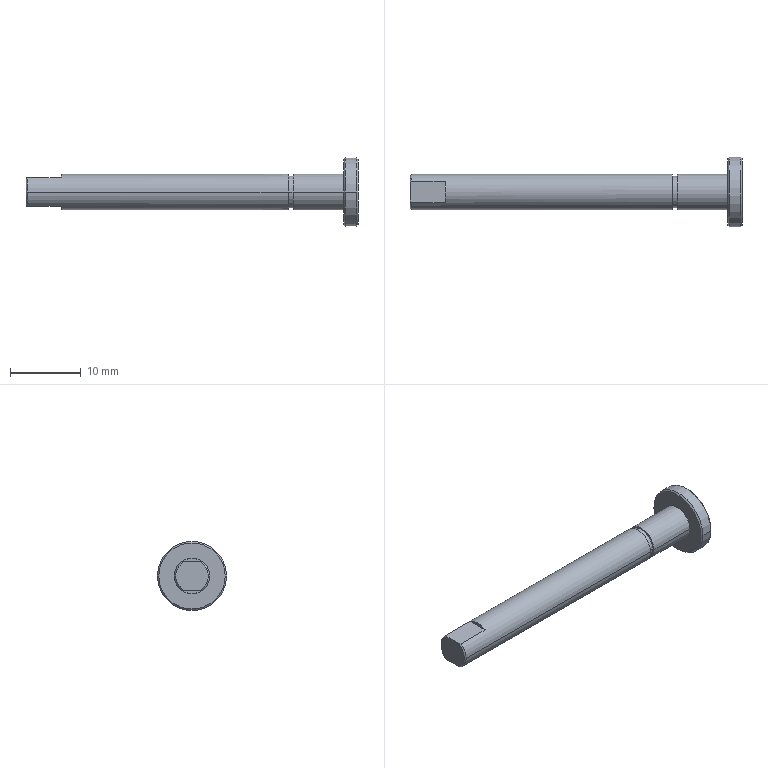Component | SolidWorks | 18MTOSC80BatteryCellCornerFoldingRollerAssembly-1_18ZTJ-NVT-01-002-1 | 1 solid | 24 faces | box 47 x 9.8 x 9.8 mm | volume 1020 mm3 | plane 9 | cylinder 8 | cone 7 | commonest cylinder face diameters 5 x4 4.5 x2 9.8 x2 | material Chrome Plated Rod
build123d program:
from build123d import *

# Parameters (mm, degrees)
SKETCH1_R           = 2.5
BOSS_EXTRUDE1_DEPTH = 45
SKETCH2_R           = 4.9
BOSS_EXTRUDE2_DEPTH = 2
CHAMFER1_SIZE       = 0.2
CUT_EXTRUDE2_START  = 0.7
SKETCH4_R           = 2.5
SKETCH4_R_2         = 2.25
CUT_EXTRUDE2_DEPTH  = 0.7
CUT_EXTRUDE3_DEPTH  = 5


with BuildPart() as part:
    # Sketch1 → Boss-Extrude1 (new body)
    with BuildSketch(Plane(origin=(0, 0, 0), x_dir=(1, 0, 0), z_dir=(0, 1, 0))):
        with Locations(Location((0, 0, 0), (0, 0, 90))):
            Circle(SKETCH1_R)
    extrude(amount=BOSS_EXTRUDE1_DEPTH)

    # Sketch2 → Boss-Extrude2 (add)
    with BuildSketch(Plane(origin=(0, 45, 0), x_dir=(1, 0, 0), z_dir=(0, 1, 0))):
        with Locations(Location((0, 0, 0), (0, 0, 270))):
            Circle(SKETCH2_R)
    extrude(amount=BOSS_EXTRUDE2_DEPTH)

    # Chamfer1
    chamfer1_edges = [part.edges().sort_by_distance(p)[0] for p in [
        (0, 0, 2.5),
        (0, 45, -4.9),
        (0, 47, -4.9),
    ]]
    chamfer(chamfer1_edges, length=CHAMFER1_SIZE)

    # Sketch4 → Cut-Extrude2 (cut)
    with BuildSketch(Plane(origin=(0, 37.8, 0), x_dir=(-1, 0, 0), z_dir=(0, -1, 0)).offset(CUT_EXTRUDE2_START)):
        with Locations(Location((0, 0, 0), (0, 0, 90))):
            Circle(SKETCH4_R)
        with Locations(Location((0, 0, 0), (0, 0, 90))):
            Circle(SKETCH4_R_2, mode=Mode.SUBTRACT)
    extrude(amount=-CUT_EXTRUDE2_DEPTH, mode=Mode.SUBTRACT)

    # Sketch5 → Cut-Extrude3 (cut)
    with BuildSketch(Plane.XZ):
        with BuildLine():
            Line((-2, 1.5), (-2, -1.5))
            ThreePointArc((-2, -1.5), (-2.5, 0), (-2, 1.5))
        make_face()
        with BuildLine():
            Line((2, 1.5), (2, -1.5))
            ThreePointArc((2, -1.5), (2.5, 0), (2, 1.5))
        make_face()
    extrude(amount=-CUT_EXTRUDE3_DEPTH, mode=Mode.SUBTRACT)


solid = part.part

# Placed as in the assembly
solid = solid.moved(Location((-30.1, -14.53, 131), (90, 0, -90)))
STEP:
#1=CARTESIAN_POINT('',(0.2756,-0.6705,5.157));
#2=VERTEX_POINT('',#1);
#3=CARTESIAN_POINT('',(0.2756,-0.4736,5.157));
#4=VERTEX_POINT('',#3);
#5=CARTESIAN_POINT('',(0.2756,-0.572,5.157));
#6=DIRECTION('',(-1.,-0.,-0.));
#7=DIRECTION('',(0.,-1.,0.));
#8=AXIS2_PLACEMENT_3D('',#5,#6,#7);
#9=CIRCLE('',#8,0.09843);
#10=EDGE_CURVE('',#2,#4,#9,.T.);
#11=ORIENTED_EDGE('',*,*,#10,.T.);
#12=CARTESIAN_POINT('',(-1.177,-0.4736,5.157));
#13=VERTEX_POINT('',#12);
#14=CARTESIAN_POINT('',(0.5866,-0.4736,5.157));
#15=DIRECTION('',(-1.,-0.,-0.));
#16=VECTOR('',#15,39.37);
#17=LINE('',#14,#16);
#18=EDGE_CURVE('',#4,#13,#17,.T.);
#19=ORIENTED_EDGE('',*,*,#18,.T.);
#20=CARTESIAN_POINT('',(-1.177,-0.513,5.236));
#21=VERTEX_POINT('',#20);
#22=CARTESIAN_POINT('',(-1.177,-0.572,5.157));
#23=DIRECTION('',(1.,0.,0.));
#24=DIRECTION('',(0.,1.,0.));
#25=AXIS2_PLACEMENT_3D('',#22,#23,#24);
#26=CIRCLE('',#25,0.09843);
#27=EDGE_CURVE('',#13,#21,#26,.T.);
#28=ORIENTED_EDGE('',*,*,#27,.T.);
#29=CARTESIAN_POINT('',(-0.9882,-0.513,5.236));
#30=VERTEX_POINT('',#29);
#31=CARTESIAN_POINT('',(-0.9882,-0.513,5.236));
#32=DIRECTION('',(-1.,-0.,-0.));
#33=VECTOR('',#32,39.37);
#34=LINE('',#31,#33);
#35=EDGE_CURVE('',#30,#21,#34,.T.);
#36=ORIENTED_EDGE('',*,*,#35,.F.);
#37=CARTESIAN_POINT('',(-0.9882,-0.6311,5.236));
#38=VERTEX_POINT('',#37);
#39=CARTESIAN_POINT('',(-0.9882,-0.572,5.157));
#40=DIRECTION('',(-1.,-0.,-0.));
#41=DIRECTION('',(0.,-1.,0.));
#42=AXIS2_PLACEMENT_3D('',#39,#40,#41);
#43=CIRCLE('',#42,0.09843);
#44=EDGE_CURVE('',#38,#30,#43,.T.);
#45=ORIENTED_EDGE('',*,*,#44,.F.);
#46=CARTESIAN_POINT('',(-1.177,-0.6311,5.236));
#47=VERTEX_POINT('',#46);
#48=CARTESIAN_POINT('',(-0.9882,-0.6311,5.236));
#49=DIRECTION('',(-1.,-0.,-0.));
#50=VECTOR('',#49,39.37);
#51=LINE('',#48,#50);
#52=EDGE_CURVE('',#38,#47,#51,.T.);
#53=ORIENTED_EDGE('',*,*,#52,.T.);
#54=CARTESIAN_POINT('',(-1.177,-0.6705,5.157));
#55=VERTEX_POINT('',#54);
#56=CARTESIAN_POINT('',(-1.177,-0.572,5.157));
#57=DIRECTION('',(1.,0.,0.));
#58=DIRECTION('',(0.,1.,0.));
#59=AXIS2_PLACEMENT_3D('',#56,#57,#58);
#60=CIRCLE('',#59,0.09843);
#61=EDGE_CURVE('',#47,#55,#60,.T.);
#62=ORIENTED_EDGE('',*,*,#61,.T.);
#63=CARTESIAN_POINT('',(0.5866,-0.6705,5.157));
#64=DIRECTION('',(-1.,-0.,-0.));
#65=VECTOR('',#64,39.37);
#66=LINE('',#63,#65);
#67=EDGE_CURVE('',#2,#55,#66,.T.);
#68=ORIENTED_EDGE('',*,*,#67,.F.);
#69=EDGE_LOOP('',(#11,#19,#28,#36,#45,#53,#62,#68));
#70=FACE_OUTER_BOUND('',#69,.T.);
#71=CARTESIAN_POINT('',(0.5866,-0.572,5.157));
#72=DIRECTION('',(-1.,-0.,-0.));
#73=DIRECTION('',(0.,-1.,0.));
#74=AXIS2_PLACEMENT_3D('',#71,#72,#73);
#75=CYLINDRICAL_SURFACE('',#74,0.09843);
#76=ADVANCED_FACE('',(#70),#75,.T.);
#77=CARTESIAN_POINT('',(-1.185,-0.4815,5.157));
#78=VERTEX_POINT('',#77);
#79=CARTESIAN_POINT('',(-1.185,-0.5273,5.079));
#80=VERTEX_POINT('',#79);
#81=CARTESIAN_POINT('',(-1.185,-0.572,5.157));
#82=DIRECTION('',(-1.,-0.,-0.));
#83=DIRECTION('',(0.,1.,0.));
#84=AXIS2_PLACEMENT_3D('',#81,#82,#83);
#85=CIRCLE('',#84,0.09055);
#86=EDGE_CURVE('',#78,#80,#85,.T.);
#87=ORIENTED_EDGE('',*,*,#86,.F.);
#88=CARTESIAN_POINT('',(-1.177,-0.4736,5.157));
#89=DIRECTION('',(0.7071,0.7071,0.));
#90=VECTOR('',#89,39.37);
#91=LINE('',#88,#90);
#92=EDGE_CURVE('',#78,#13,#91,.T.);
#93=ORIENTED_EDGE('',*,*,#92,.T.);
#94=CARTESIAN_POINT('',(-1.177,-0.513,5.079));
#95=VERTEX_POINT('',#94);
#96=CARTESIAN_POINT('',(-1.177,-0.572,5.157));
#97=DIRECTION('',(1.,0.,0.));
#98=DIRECTION('',(0.,1.,0.));
#99=AXIS2_PLACEMENT_3D('',#96,#97,#98);
#100=CIRCLE('',#99,0.09843);
#101=EDGE_CURVE('',#95,#13,#100,.T.);
#102=ORIENTED_EDGE('',*,*,#101,.F.);
#103=CARTESIAN_POINT('',(-1.185,-0.5273,5.079));
#104=CARTESIAN_POINT('',(-1.183,-0.5224,5.079));
#105=CARTESIAN_POINT('',(-1.18,-0.5176,5.079));
#106=CARTESIAN_POINT('',(-1.177,-0.513,5.079));
#107=B_SPLINE_CURVE_WITH_KNOTS('',3,(#103,#104,#105,#106),.UNSPECIFIED.,.F.,.F.,(4,4),(0.005045,0.005461),.UNSPECIFIED.);
#108=EDGE_CURVE('',#80,#95,#107,.T.);
#109=ORIENTED_EDGE('',*,*,#108,.F.);
#110=EDGE_LOOP('',(#87,#93,#102,#109));
#111=FACE_OUTER_BOUND('',#110,.T.);
#112=CARTESIAN_POINT('',(-1.177,-0.572,5.157));
#113=DIRECTION('',(1.,0.,0.));
#114=DIRECTION('',(0.,1.,0.));
#115=AXIS2_PLACEMENT_3D('',#112,#113,#114);
#116=CONICAL_SURFACE('',#115,0.09843,0.7854);
#117=ADVANCED_FACE('',(#111),#116,.T.);
#118=CARTESIAN_POINT('',(0.2756,-0.6606,5.157));
#119=VERTEX_POINT('',#118);
#120=CARTESIAN_POINT('',(0.2756,-0.4835,5.157));
#121=VERTEX_POINT('',#120);
#122=CARTESIAN_POINT('',(0.2756,-0.572,5.157));
#123=DIRECTION('',(-1.,-0.,-0.));
#124=DIRECTION('',(0.,-1.,0.));
#125=AXIS2_PLACEMENT_3D('',#122,#123,#124);
#126=CIRCLE('',#125,0.08858);
#127=EDGE_CURVE('',#119,#121,#126,.T.);
#128=ORIENTED_EDGE('',*,*,#127,.F.);
#129=CARTESIAN_POINT('',(0.3032,-0.6606,5.157));
#130=VERTEX_POINT('',#129);
#131=CARTESIAN_POINT('',(0.2756,-0.6606,5.157));
#132=DIRECTION('',(1.,0.,0.));
#133=VECTOR('',#132,39.37);
#134=LINE('',#131,#133);
#135=EDGE_CURVE('',#119,#130,#134,.T.);
#136=ORIENTED_EDGE('',*,*,#135,.T.);
#137=CARTESIAN_POINT('',(0.3032,-0.4835,5.157));
#138=VERTEX_POINT('',#137);
#139=CARTESIAN_POINT('',(0.3032,-0.572,5.157));
#140=DIRECTION('',(-1.,-0.,-0.));
#141=DIRECTION('',(0.,-1.,0.));
#142=AXIS2_PLACEMENT_3D('',#139,#140,#141);
#143=CIRCLE('',#142,0.08858);
#144=EDGE_CURVE('',#130,#138,#143,.T.);
#145=ORIENTED_EDGE('',*,*,#144,.T.);
#146=CARTESIAN_POINT('',(0.2756,-0.4835,5.157));
#147=DIRECTION('',(1.,0.,0.));
#148=VECTOR('',#147,39.37);
#149=LINE('',#146,#148);
#150=EDGE_CURVE('',#121,#138,#149,.T.);
#151=ORIENTED_EDGE('',*,*,#150,.F.);
#152=EDGE_LOOP('',(#128,#136,#145,#151));
#153=FACE_OUTER_BOUND('',#152,.T.);
#154=CARTESIAN_POINT('',(0.2756,-0.572,5.157));
#155=DIRECTION('',(1.,0.,0.));
#156=DIRECTION('',(0.,1.,0.));
#157=AXIS2_PLACEMENT_3D('',#154,#155,#156);
#158=CYLINDRICAL_SURFACE('',#157,0.08858);
#159=ADVANCED_FACE('',(#153),#158,.T.);
#160=CARTESIAN_POINT('',(0.6654,-0.387,5.157));
#161=VERTEX_POINT('',#160);
#162=CARTESIAN_POINT('',(0.6654,-0.7571,5.157));
#163=VERTEX_POINT('',#162);
#164=CARTESIAN_POINT('',(0.6654,-0.572,5.157));
#165=DIRECTION('',(1.,0.,0.));
#166=DIRECTION('',(0.,1.,0.));
#167=AXIS2_PLACEMENT_3D('',#164,#165,#166);
#168=CIRCLE('',#167,0.185);
#169=EDGE_CURVE('',#161,#163,#168,.T.);
#170=ORIENTED_EDGE('',*,*,#169,.F.);
#171=CARTESIAN_POINT('',(0.6575,-0.3791,5.157));
#172=VERTEX_POINT('',#171);
#173=CARTESIAN_POINT('',(0.6654,-0.387,5.157));
#174=DIRECTION('',(-0.7071,0.7071,0.));
#175=VECTOR('',#174,39.37);
#176=LINE('',#173,#175);
#177=EDGE_CURVE('',#161,#172,#176,.T.);
#178=ORIENTED_EDGE('',*,*,#177,.T.);
#179=CARTESIAN_POINT('',(0.6575,-0.765,5.157));
#180=VERTEX_POINT('',#179);
#181=CARTESIAN_POINT('',(0.6575,-0.572,5.157));
#182=DIRECTION('',(-1.,-0.,-0.));
#183=DIRECTION('',(0.,1.,0.));
#184=AXIS2_PLACEMENT_3D('',#181,#182,#183);
#185=CIRCLE('',#184,0.1929);
#186=EDGE_CURVE('',#180,#172,#185,.T.);
#187=ORIENTED_EDGE('',*,*,#186,.F.);
#188=CARTESIAN_POINT('',(0.6654,-0.7571,5.157));
#189=DIRECTION('',(-0.7071,-0.7071,-0.));
#190=VECTOR('',#189,39.37);
#191=LINE('',#188,#190);
#192=EDGE_CURVE('',#163,#180,#191,.T.);
#193=ORIENTED_EDGE('',*,*,#192,.F.);
#194=EDGE_LOOP('',(#170,#178,#187,#193));
#195=FACE_OUTER_BOUND('',#194,.T.);
#196=CARTESIAN_POINT('',(0.6654,-0.572,5.157));
#197=DIRECTION('',(-1.,-0.,-0.));
#198=DIRECTION('',(0.,-1.,0.));
#199=AXIS2_PLACEMENT_3D('',#196,#197,#198);
#200=CONICAL_SURFACE('',#199,0.185,0.7854);
#201=ADVANCED_FACE('',(#195),#200,.T.);
#202=CARTESIAN_POINT('',(0.5866,-0.7571,5.157));
#203=VERTEX_POINT('',#202);
#204=CARTESIAN_POINT('',(0.5866,-0.387,5.157));
#205=VERTEX_POINT('',#204);
#206=CARTESIAN_POINT('',(0.5866,-0.572,5.157));
#207=DIRECTION('',(-1.,-0.,-0.));
#208=DIRECTION('',(0.,1.,0.));
#209=AXIS2_PLACEMENT_3D('',#206,#207,#208);
#210=CIRCLE('',#209,0.185);
#211=EDGE_CURVE('',#203,#205,#210,.T.);
#212=ORIENTED_EDGE('',*,*,#211,.F.);
#213=CARTESIAN_POINT('',(0.5945,-0.765,5.157));
#214=VERTEX_POINT('',#213);
#215=CARTESIAN_POINT('',(0.5945,-0.765,5.157));
#216=DIRECTION('',(0.7071,-0.7071,0.));
#217=VECTOR('',#216,39.37);
#218=LINE('',#215,#217);
#219=EDGE_CURVE('',#203,#214,#218,.T.);
#220=ORIENTED_EDGE('',*,*,#219,.T.);
#221=CARTESIAN_POINT('',(0.5945,-0.3791,5.157));
#222=VERTEX_POINT('',#221);
#223=CARTESIAN_POINT('',(0.5945,-0.572,5.157));
#224=DIRECTION('',(1.,0.,0.));
#225=DIRECTION('',(-0.,1.,0.));
#226=AXIS2_PLACEMENT_3D('',#223,#224,#225);
#227=CIRCLE('',#226,0.1929);
#228=EDGE_CURVE('',#222,#214,#227,.T.);
#229=ORIENTED_EDGE('',*,*,#228,.F.);
#230=CARTESIAN_POINT('',(0.5945,-0.3791,5.157));
#231=DIRECTION('',(0.7071,0.7071,0.));
#232=VECTOR('',#231,39.37);
#233=LINE('',#230,#232);
#234=EDGE_CURVE('',#205,#222,#233,.T.);
#235=ORIENTED_EDGE('',*,*,#234,.F.);
#236=EDGE_LOOP('',(#212,#220,#229,#235));
#237=FACE_OUTER_BOUND('',#236,.T.);
#238=CARTESIAN_POINT('',(0.5945,-0.572,5.157));
#239=DIRECTION('',(1.,0.,0.));
#240=DIRECTION('',(-0.,1.,0.));
#241=AXIS2_PLACEMENT_3D('',#238,#239,#240);
#242=CONICAL_SURFACE('',#241,0.1929,0.7854);
#243=ADVANCED_FACE('',(#237),#242,.T.);
#244=ORIENTED_EDGE('',*,*,#186,.T.);
#245=CARTESIAN_POINT('',(0.6654,-0.3791,5.157));
#246=DIRECTION('',(-1.,-0.,-0.));
#247=VECTOR('',#246,39.37);
#248=LINE('',#245,#247);
#249=EDGE_CURVE('',#172,#222,#248,.T.);
#250=ORIENTED_EDGE('',*,*,#249,.T.);
#251=ORIENTED_EDGE('',*,*,#228,.T.);
#252=CARTESIAN_POINT('',(0.6654,-0.765,5.157));
#253=DIRECTION('',(-1.,-0.,-0.));
#254=VECTOR('',#253,39.37);
#255=LINE('',#252,#254);
#256=EDGE_CURVE('',#180,#214,#255,.T.);
#257=ORIENTED_EDGE('',*,*,#256,.F.);
#258=EDGE_LOOP('',(#244,#250,#251,#257));
#259=FACE_OUTER_BOUND('',#258,.T.);
#260=CARTESIAN_POINT('',(0.6654,-0.572,5.157));
#261=DIRECTION('',(-1.,-0.,-0.));
#262=DIRECTION('',(0.,-1.,0.));
#263=AXIS2_PLACEMENT_3D('',#260,#261,#262);
#264=CYLINDRICAL_SURFACE('',#263,0.1929);
#265=ADVANCED_FACE('',(#259),#264,.T.);
#266=CARTESIAN_POINT('',(0.5866,-0.4736,5.157));
#267=VERTEX_POINT('',#266);
#268=CARTESIAN_POINT('',(0.5866,-0.6705,5.157));
#269=VERTEX_POINT('',#268);
#270=CARTESIAN_POINT('',(0.5866,-0.572,5.157));
#271=DIRECTION('',(1.,0.,0.));
#272=DIRECTION('',(0.,1.,0.));
#273=AXIS2_PLACEMENT_3D('',#270,#271,#272);
#274=CIRCLE('',#273,0.09843);
#275=EDGE_CURVE('',#267,#269,#274,.T.);
#276=ORIENTED_EDGE('',*,*,#275,.F.);
#277=CARTESIAN_POINT('',(0.3032,-0.4736,5.157));
#278=VERTEX_POINT('',#277);
#279=CARTESIAN_POINT('',(0.5866,-0.4736,5.157));
#280=DIRECTION('',(-1.,-0.,-0.));
#281=VECTOR('',#280,39.37);
#282=LINE('',#279,#281);
#283=EDGE_CURVE('',#267,#278,#282,.T.);
#284=ORIENTED_EDGE('',*,*,#283,.T.);
#285=CARTESIAN_POINT('',(0.3032,-0.6705,5.157));
#286=VERTEX_POINT('',#285);
#287=CARTESIAN_POINT('',(0.3032,-0.572,5.157));
#288=DIRECTION('',(-1.,-0.,-0.));
#289=DIRECTION('',(0.,-1.,0.));
#290=AXIS2_PLACEMENT_3D('',#287,#288,#289);
#291=CIRCLE('',#290,0.09843);
#292=EDGE_CURVE('',#286,#278,#291,.T.);
#293=ORIENTED_EDGE('',*,*,#292,.F.);
#294=CARTESIAN_POINT('',(0.5866,-0.6705,5.157));
#295=DIRECTION('',(-1.,-0.,-0.));
#296=VECTOR('',#295,39.37);
#297=LINE('',#294,#296);
#298=EDGE_CURVE('',#269,#286,#297,.T.);
#299=ORIENTED_EDGE('',*,*,#298,.F.);
#300=EDGE_LOOP('',(#276,#284,#293,#299));
#301=FACE_OUTER_BOUND('',#300,.T.);
#302=CARTESIAN_POINT('',(0.5866,-0.572,5.157));
#303=DIRECTION('',(-1.,-0.,-0.));
#304=DIRECTION('',(0.,-1.,0.));
#305=AXIS2_PLACEMENT_3D('',#302,#303,#304);
#306=CYLINDRICAL_SURFACE('',#305,0.09843);
#307=ADVANCED_FACE('',(#301),#306,.T.);
#308=CARTESIAN_POINT('',(-1.177,-0.6311,5.079));
#309=VERTEX_POINT('',#308);
#310=CARTESIAN_POINT('',(-1.185,-0.6168,5.079));
#311=VERTEX_POINT('',#310);
#312=CARTESIAN_POINT('',(-1.177,-0.6311,5.079));
#313=CARTESIAN_POINT('',(-1.18,-0.6264,5.079));
#314=CARTESIAN_POINT('',(-1.183,-0.6216,5.079));
#315=CARTESIAN_POINT('',(-1.185,-0.6168,5.079));
#316=B_SPLINE_CURVE_WITH_KNOTS('',3,(#312,#313,#314,#315),.UNSPECIFIED.,.F.,.F.,(4,4),(0.002264,0.002682),.UNSPECIFIED.);
#317=EDGE_CURVE('',#309,#311,#316,.T.);
#318=ORIENTED_EDGE('',*,*,#317,.F.);
#319=CARTESIAN_POINT('',(-1.177,-0.572,5.157));
#320=DIRECTION('',(1.,0.,0.));
#321=DIRECTION('',(0.,1.,0.));
#322=AXIS2_PLACEMENT_3D('',#319,#320,#321);
#323=CIRCLE('',#322,0.09843);
#324=EDGE_CURVE('',#55,#309,#323,.T.);
#325=ORIENTED_EDGE('',*,*,#324,.F.);
#326=ORIENTED_EDGE('',*,*,#61,.F.);
#327=CARTESIAN_POINT('',(-1.185,-0.6168,5.236));
#328=VERTEX_POINT('',#327);
#329=CARTESIAN_POINT('',(-1.185,-0.6168,5.236));
#330=CARTESIAN_POINT('',(-1.183,-0.6217,5.236));
#331=CARTESIAN_POINT('',(-1.18,-0.6264,5.236));
#332=CARTESIAN_POINT('',(-1.177,-0.6311,5.236));
#333=B_SPLINE_CURVE_WITH_KNOTS('',3,(#329,#330,#331,#332),.UNSPECIFIED.,.F.,.F.,(4,4),(0.005045,0.005461),.UNSPECIFIED.);
#334=EDGE_CURVE('',#328,#47,#333,.T.);
#335=ORIENTED_EDGE('',*,*,#334,.F.);
#336=CARTESIAN_POINT('',(-1.185,-0.572,5.157));
#337=DIRECTION('',(-1.,-0.,-0.));
#338=DIRECTION('',(0.,1.,0.));
#339=AXIS2_PLACEMENT_3D('',#336,#337,#338);
#340=CIRCLE('',#339,0.09055);
#341=EDGE_CURVE('',#311,#328,#340,.T.);
#342=ORIENTED_EDGE('',*,*,#341,.F.);
#343=EDGE_LOOP('',(#318,#325,#326,#335,#342));
#344=FACE_OUTER_BOUND('',#343,.T.);
#345=CARTESIAN_POINT('',(-1.177,-0.572,5.157));
#346=DIRECTION('',(1.,0.,0.));
#347=DIRECTION('',(0.,1.,0.));
#348=AXIS2_PLACEMENT_3D('',#345,#346,#347);
#349=CONICAL_SURFACE('',#348,0.09843,0.7854);
#350=ADVANCED_FACE('',(#344),#349,.T.);
#351=ORIENTED_EDGE('',*,*,#283,.F.);
#352=CARTESIAN_POINT('',(0.5866,-0.572,5.157));
#353=DIRECTION('',(1.,0.,0.));
#354=DIRECTION('',(0.,1.,0.));
#355=AXIS2_PLACEMENT_3D('',#352,#353,#354);
#356=CIRCLE('',#355,0.09843);
#357=EDGE_CURVE('',#269,#267,#356,.T.);
#358=ORIENTED_EDGE('',*,*,#357,.F.);
#359=ORIENTED_EDGE('',*,*,#298,.T.);
#360=CARTESIAN_POINT('',(0.3032,-0.572,5.157));
#361=DIRECTION('',(-1.,-0.,-0.));
#362=DIRECTION('',(0.,-1.,0.));
#363=AXIS2_PLACEMENT_3D('',#360,#361,#362);
#364=CIRCLE('',#363,0.09843);
#365=EDGE_CURVE('',#278,#286,#364,.T.);
#366=ORIENTED_EDGE('',*,*,#365,.F.);
#367=EDGE_LOOP('',(#351,#358,#359,#366));
#368=FACE_OUTER_BOUND('',#367,.T.);
#369=CARTESIAN_POINT('',(0.5866,-0.572,5.157));
#370=DIRECTION('',(-1.,-0.,-0.));
#371=DIRECTION('',(0.,-1.,0.));
#372=AXIS2_PLACEMENT_3D('',#369,#370,#371);
#373=CYLINDRICAL_SURFACE('',#372,0.09843);
#374=ADVANCED_FACE('',(#368),#373,.T.);
#375=ORIENTED_EDGE('',*,*,#249,.F.);
#376=CARTESIAN_POINT('',(0.6575,-0.572,5.157));
#377=DIRECTION('',(-1.,-0.,-0.));
#378=DIRECTION('',(0.,1.,0.));
#379=AXIS2_PLACEMENT_3D('',#376,#377,#378);
#380=CIRCLE('',#379,0.1929);
#381=EDGE_CURVE('',#172,#180,#380,.T.);
#382=ORIENTED_EDGE('',*,*,#381,.T.);
#383=ORIENTED_EDGE('',*,*,#256,.T.);
#384=CARTESIAN_POINT('',(0.5945,-0.572,5.157));
#385=DIRECTION('',(1.,0.,0.));
#386=DIRECTION('',(-0.,1.,0.));
#387=AXIS2_PLACEMENT_3D('',#384,#385,#386);
#388=CIRCLE('',#387,0.1929);
#389=EDGE_CURVE('',#214,#222,#388,.T.);
#390=ORIENTED_EDGE('',*,*,#389,.T.);
#391=EDGE_LOOP('',(#375,#382,#383,#390));
#392=FACE_OUTER_BOUND('',#391,.T.);
#393=CARTESIAN_POINT('',(0.6654,-0.572,5.157));
#394=DIRECTION('',(-1.,-0.,-0.));
#395=DIRECTION('',(0.,-1.,0.));
#396=AXIS2_PLACEMENT_3D('',#393,#394,#395);
#397=CYLINDRICAL_SURFACE('',#396,0.1929);
#398=ADVANCED_FACE('',(#392),#397,.T.);
#399=CARTESIAN_POINT('',(0.6654,-0.572,5.157));
#400=DIRECTION('',(1.,0.,0.));
#401=DIRECTION('',(0.,1.,0.));
#402=AXIS2_PLACEMENT_3D('',#399,#400,#401);
#403=CIRCLE('',#402,0.185);
#404=EDGE_CURVE('',#163,#161,#403,.T.);
#405=ORIENTED_EDGE('',*,*,#404,.T.);
#406=ORIENTED_EDGE('',*,*,#169,.T.);
#407=EDGE_LOOP('',(#405,#406));
#408=FACE_OUTER_BOUND('',#407,.T.);
#409=CARTESIAN_POINT('',(0.6654,-0.572,5.157));
#410=DIRECTION('',(1.,0.,0.));
#411=DIRECTION('',(-0.,1.,-0.));
#412=AXIS2_PLACEMENT_3D('',#409,#410,#411);
#413=PLANE('',#412);
#414=ADVANCED_FACE('',(#408),#413,.T.);
#415=CARTESIAN_POINT('',(0.5866,-0.572,5.157));
#416=DIRECTION('',(-1.,-0.,-0.));
#417=DIRECTION('',(0.,1.,0.));
#418=AXIS2_PLACEMENT_3D('',#415,#416,#417);
#419=CIRCLE('',#418,0.185);
#420=EDGE_CURVE('',#205,#203,#419,.T.);
#421=ORIENTED_EDGE('',*,*,#420,.T.);
#422=ORIENTED_EDGE('',*,*,#211,.T.);
#423=EDGE_LOOP('',(#421,#422));
#424=FACE_OUTER_BOUND('',#423,.T.);
#425=ORIENTED_EDGE('',*,*,#357,.T.);
#426=ORIENTED_EDGE('',*,*,#275,.T.);
#427=EDGE_LOOP('',(#425,#426));
#428=FACE_BOUND('',#427,.T.);
#429=CARTESIAN_POINT('',(0.5866,-0.572,5.157));
#430=DIRECTION('',(1.,0.,0.));
#431=DIRECTION('',(-0.,1.,-0.));
#432=AXIS2_PLACEMENT_3D('',#429,#430,#431);
#433=PLANE('',#432);
#434=ADVANCED_FACE('',(#424,#428),#433,.F.);
#435=ORIENTED_EDGE('',*,*,#219,.F.);
#436=ORIENTED_EDGE('',*,*,#420,.F.);
#437=ORIENTED_EDGE('',*,*,#234,.T.);
#438=ORIENTED_EDGE('',*,*,#389,.F.);
#439=EDGE_LOOP('',(#435,#436,#437,#438));
#440=FACE_OUTER_BOUND('',#439,.T.);
#441=CARTESIAN_POINT('',(0.5945,-0.572,5.157));
#442=DIRECTION('',(1.,0.,0.));
#443=DIRECTION('',(-0.,1.,0.));
#444=AXIS2_PLACEMENT_3D('',#441,#442,#443);
#445=CONICAL_SURFACE('',#444,0.1929,0.7854);
#446=ADVANCED_FACE('',(#440),#445,.T.);
#447=ORIENTED_EDGE('',*,*,#177,.F.);
#448=ORIENTED_EDGE('',*,*,#404,.F.);
#449=ORIENTED_EDGE('',*,*,#192,.T.);
#450=ORIENTED_EDGE('',*,*,#381,.F.);
#451=EDGE_LOOP('',(#447,#448,#449,#450));
#452=FACE_OUTER_BOUND('',#451,.T.);
#453=CARTESIAN_POINT('',(0.6654,-0.572,5.157));
#454=DIRECTION('',(-1.,-0.,-0.));
#455=DIRECTION('',(0.,-1.,0.));
#456=AXIS2_PLACEMENT_3D('',#453,#454,#455);
#457=CONICAL_SURFACE('',#456,0.185,0.7854);
#458=ADVANCED_FACE('',(#452),#457,.T.);
#459=ORIENTED_EDGE('',*,*,#10,.F.);
#460=CARTESIAN_POINT('',(0.2756,-0.572,5.157));
#461=DIRECTION('',(-1.,-0.,-0.));
#462=DIRECTION('',(0.,-1.,0.));
#463=AXIS2_PLACEMENT_3D('',#460,#461,#462);
#464=CIRCLE('',#463,0.09843);
#465=EDGE_CURVE('',#4,#2,#464,.T.);
#466=ORIENTED_EDGE('',*,*,#465,.F.);
#467=EDGE_LOOP('',(#459,#466));
#468=FACE_OUTER_BOUND('',#467,.T.);
#469=CARTESIAN_POINT('',(0.2756,-0.572,5.157));
#470=DIRECTION('',(-1.,-0.,-0.));
#471=DIRECTION('',(0.,-1.,0.));
#472=AXIS2_PLACEMENT_3D('',#469,#470,#471);
#473=CIRCLE('',#472,0.08858);
#474=EDGE_CURVE('',#121,#119,#473,.T.);
#475=ORIENTED_EDGE('',*,*,#474,.T.);
#476=ORIENTED_EDGE('',*,*,#127,.T.);
#477=EDGE_LOOP('',(#475,#476));
#478=FACE_BOUND('',#477,.T.);
#479=CARTESIAN_POINT('',(0.2756,-0.572,5.157));
#480=DIRECTION('',(-1.,-0.,-0.));
#481=DIRECTION('',(0.,-1.,0.));
#482=AXIS2_PLACEMENT_3D('',#479,#480,#481);
#483=PLANE('',#482);
#484=ADVANCED_FACE('',(#468,#478),#483,.F.);
#485=ORIENTED_EDGE('',*,*,#292,.T.);
#486=ORIENTED_EDGE('',*,*,#365,.T.);
#487=EDGE_LOOP('',(#485,#486));
#488=FACE_OUTER_BOUND('',#487,.T.);
#489=CARTESIAN_POINT('',(0.3032,-0.572,5.157));
#490=DIRECTION('',(-1.,-0.,-0.));
#491=DIRECTION('',(0.,-1.,0.));
#492=AXIS2_PLACEMENT_3D('',#489,#490,#491);
#493=CIRCLE('',#492,0.08858);
#494=EDGE_CURVE('',#138,#130,#493,.T.);
#495=ORIENTED_EDGE('',*,*,#494,.F.);
#496=ORIENTED_EDGE('',*,*,#144,.F.);
#497=EDGE_LOOP('',(#495,#496));
#498=FACE_BOUND('',#497,.T.);
#499=CARTESIAN_POINT('',(0.3032,-0.572,5.157));
#500=DIRECTION('',(-1.,-0.,-0.));
#501=DIRECTION('',(0.,-1.,0.));
#502=AXIS2_PLACEMENT_3D('',#499,#500,#501);
#503=PLANE('',#502);
#504=ADVANCED_FACE('',(#488,#498),#503,.T.);
#505=ORIENTED_EDGE('',*,*,#135,.F.);
#506=ORIENTED_EDGE('',*,*,#474,.F.);
#507=ORIENTED_EDGE('',*,*,#150,.T.);
#508=ORIENTED_EDGE('',*,*,#494,.T.);
#509=EDGE_LOOP('',(#505,#506,#507,#508));
#510=FACE_OUTER_BOUND('',#509,.T.);
#511=CARTESIAN_POINT('',(0.2756,-0.572,5.157));
#512=DIRECTION('',(1.,0.,0.));
#513=DIRECTION('',(0.,1.,0.));
#514=AXIS2_PLACEMENT_3D('',#511,#512,#513);
#515=CYLINDRICAL_SURFACE('',#514,0.08858);
#516=ADVANCED_FACE('',(#510),#515,.T.);
#517=CARTESIAN_POINT('',(-1.185,-0.5273,5.236));
#518=VERTEX_POINT('',#517);
#519=CARTESIAN_POINT('',(-1.185,-0.572,5.157));
#520=DIRECTION('',(-1.,-0.,-0.));
#521=DIRECTION('',(0.,1.,0.));
#522=AXIS2_PLACEMENT_3D('',#519,#520,#521);
#523=CIRCLE('',#522,0.09055);
#524=EDGE_CURVE('',#518,#78,#523,.T.);
#525=ORIENTED_EDGE('',*,*,#524,.T.);
#526=ORIENTED_EDGE('',*,*,#86,.T.);
#527=CARTESIAN_POINT('',(-1.185,-0.513,5.079));
#528=DIRECTION('',(-0.,1.,-0.));
#529=VECTOR('',#528,39.37);
#530=LINE('',#527,#529);
#531=EDGE_CURVE('',#311,#80,#530,.T.);
#532=ORIENTED_EDGE('',*,*,#531,.F.);
#533=ORIENTED_EDGE('',*,*,#341,.T.);
#534=CARTESIAN_POINT('',(-1.185,-0.513,5.236));
#535=DIRECTION('',(0.,-1.,0.));
#536=VECTOR('',#535,39.37);
#537=LINE('',#534,#536);
#538=EDGE_CURVE('',#518,#328,#537,.T.);
#539=ORIENTED_EDGE('',*,*,#538,.F.);
#540=EDGE_LOOP('',(#525,#526,#532,#533,#539));
#541=FACE_OUTER_BOUND('',#540,.T.);
#542=CARTESIAN_POINT('',(-1.185,-0.572,5.157));
#543=DIRECTION('',(1.,0.,0.));
#544=DIRECTION('',(-0.,1.,-0.));
#545=AXIS2_PLACEMENT_3D('',#542,#543,#544);
#546=PLANE('',#545);
#547=ADVANCED_FACE('',(#541),#546,.F.);
#548=ORIENTED_EDGE('',*,*,#92,.F.);
#549=ORIENTED_EDGE('',*,*,#524,.F.);
#550=CARTESIAN_POINT('',(-1.177,-0.513,5.236));
#551=CARTESIAN_POINT('',(-1.18,-0.5177,5.236));
#552=CARTESIAN_POINT('',(-1.183,-0.5224,5.236));
#553=CARTESIAN_POINT('',(-1.185,-0.5273,5.236));
#554=B_SPLINE_CURVE_WITH_KNOTS('',3,(#550,#551,#552,#553),.UNSPECIFIED.,.F.,.F.,(4,4),(0.002264,0.002682),.UNSPECIFIED.);
#555=EDGE_CURVE('',#21,#518,#554,.T.);
#556=ORIENTED_EDGE('',*,*,#555,.F.);
#557=ORIENTED_EDGE('',*,*,#27,.F.);
#558=EDGE_LOOP('',(#548,#549,#556,#557));
#559=FACE_OUTER_BOUND('',#558,.T.);
#560=CARTESIAN_POINT('',(-1.177,-0.572,5.157));
#561=DIRECTION('',(1.,0.,0.));
#562=DIRECTION('',(0.,1.,0.));
#563=AXIS2_PLACEMENT_3D('',#560,#561,#562);
#564=CONICAL_SURFACE('',#563,0.09843,0.7854);
#565=ADVANCED_FACE('',(#559),#564,.T.);
#566=ORIENTED_EDGE('',*,*,#18,.F.);
#567=ORIENTED_EDGE('',*,*,#465,.T.);
#568=ORIENTED_EDGE('',*,*,#67,.T.);
#569=ORIENTED_EDGE('',*,*,#324,.T.);
#570=CARTESIAN_POINT('',(-0.9882,-0.6311,5.079));
#571=VERTEX_POINT('',#570);
#572=CARTESIAN_POINT('',(-0.9882,-0.6311,5.079));
#573=DIRECTION('',(-1.,-0.,-0.));
#574=VECTOR('',#573,39.37);
#575=LINE('',#572,#574);
#576=EDGE_CURVE('',#571,#309,#575,.T.);
#577=ORIENTED_EDGE('',*,*,#576,.F.);
#578=CARTESIAN_POINT('',(-0.9882,-0.513,5.079));
#579=VERTEX_POINT('',#578);
#580=CARTESIAN_POINT('',(-0.9882,-0.572,5.157));
#581=DIRECTION('',(-1.,-0.,-0.));
#582=DIRECTION('',(0.,-1.,0.));
#583=AXIS2_PLACEMENT_3D('',#580,#581,#582);
#584=CIRCLE('',#583,0.09843);
#585=EDGE_CURVE('',#579,#571,#584,.T.);
#586=ORIENTED_EDGE('',*,*,#585,.F.);
#587=CARTESIAN_POINT('',(-0.9882,-0.513,5.079));
#588=DIRECTION('',(-1.,-0.,-0.));
#589=VECTOR('',#588,39.37);
#590=LINE('',#587,#589);
#591=EDGE_CURVE('',#579,#95,#590,.T.);
#592=ORIENTED_EDGE('',*,*,#591,.T.);
#593=ORIENTED_EDGE('',*,*,#101,.T.);
#594=EDGE_LOOP('',(#566,#567,#568,#569,#577,#586,#592,#593));
#595=FACE_OUTER_BOUND('',#594,.T.);
#596=CARTESIAN_POINT('',(0.5866,-0.572,5.157));
#597=DIRECTION('',(-1.,-0.,-0.));
#598=DIRECTION('',(0.,-1.,0.));
#599=AXIS2_PLACEMENT_3D('',#596,#597,#598);
#600=CYLINDRICAL_SURFACE('',#599,0.09843);
#601=ADVANCED_FACE('',(#595),#600,.T.);
#602=ORIENTED_EDGE('',*,*,#555,.T.);
#603=ORIENTED_EDGE('',*,*,#538,.T.);
#604=ORIENTED_EDGE('',*,*,#334,.T.);
#605=ORIENTED_EDGE('',*,*,#52,.F.);
#606=CARTESIAN_POINT('',(-0.9882,-0.513,5.236));
#607=DIRECTION('',(0.,-1.,0.));
#608=VECTOR('',#607,39.37);
#609=LINE('',#606,#608);
#610=EDGE_CURVE('',#30,#38,#609,.T.);
#611=ORIENTED_EDGE('',*,*,#610,.F.);
#612=ORIENTED_EDGE('',*,*,#35,.T.);
#613=EDGE_LOOP('',(#602,#603,#604,#605,#611,#612));
#614=FACE_OUTER_BOUND('',#613,.T.);
#615=CARTESIAN_POINT('',(-0.9882,-0.513,5.236));
#616=DIRECTION('',(0.,-0.,-1.));
#617=DIRECTION('',(-0.,1.,-0.));
#618=AXIS2_PLACEMENT_3D('',#615,#616,#617);
#619=PLANE('',#618);
#620=ADVANCED_FACE('',(#614),#619,.F.);
#621=ORIENTED_EDGE('',*,*,#44,.T.);
#622=ORIENTED_EDGE('',*,*,#610,.T.);
#623=EDGE_LOOP('',(#621,#622));
#624=FACE_OUTER_BOUND('',#623,.T.);
#625=CARTESIAN_POINT('',(-0.9882,-0.572,5.157));
#626=DIRECTION('',(-1.,-0.,-0.));
#627=DIRECTION('',(0.,-1.,0.));
#628=AXIS2_PLACEMENT_3D('',#625,#626,#627);
#629=PLANE('',#628);
#630=ADVANCED_FACE('',(#624),#629,.T.);
#631=ORIENTED_EDGE('',*,*,#317,.T.);
#632=ORIENTED_EDGE('',*,*,#531,.T.);
#633=ORIENTED_EDGE('',*,*,#108,.T.);
#634=ORIENTED_EDGE('',*,*,#591,.F.);
#635=CARTESIAN_POINT('',(-0.9882,-0.513,5.079));
#636=DIRECTION('',(-0.,1.,-0.));
#637=VECTOR('',#636,39.37);
#638=LINE('',#635,#637);
#639=EDGE_CURVE('',#571,#579,#638,.T.);
#640=ORIENTED_EDGE('',*,*,#639,.F.);
#641=ORIENTED_EDGE('',*,*,#576,.T.);
#642=EDGE_LOOP('',(#631,#632,#633,#634,#640,#641));
#643=FACE_OUTER_BOUND('',#642,.T.);
#644=CARTESIAN_POINT('',(-0.9882,-0.513,5.079));
#645=DIRECTION('',(-0.,0.,1.));
#646=DIRECTION('',(0.,-1.,0.));
#647=AXIS2_PLACEMENT_3D('',#644,#645,#646);
#648=PLANE('',#647);
#649=ADVANCED_FACE('',(#643),#648,.F.);
#650=ORIENTED_EDGE('',*,*,#585,.T.);
#651=ORIENTED_EDGE('',*,*,#639,.T.);
#652=EDGE_LOOP('',(#650,#651));
#653=FACE_OUTER_BOUND('',#652,.T.);
#654=CARTESIAN_POINT('',(-0.9882,-0.572,5.157));
#655=DIRECTION('',(-1.,-0.,-0.));
#656=DIRECTION('',(0.,-1.,0.));
#657=AXIS2_PLACEMENT_3D('',#654,#655,#656);
#658=PLANE('',#657);
#659=ADVANCED_FACE('',(#653),#658,.T.);
#660=CLOSED_SHELL('',(#76,#117,#159,#201,#243,#265,#307,#350,#374,#398,#414,#434,#446,#458,#484,#504,#516,#547,#565,#601,#620,#630,#649,#659));
#661=MANIFOLD_SOLID_BREP('',#660);
#662=CARTESIAN_POINT('',(0.,0.,0.));
#663=DIRECTION('',(0.,0.,1.));
#664=DIRECTION('',(1.,0.,0.));
#665=AXIS2_PLACEMENT_3D('',#662,#663,#664);
#666=(LENGTH_UNIT()NAMED_UNIT(*)SI_UNIT($,.METRE.));
#667=LENGTH_MEASURE_WITH_UNIT(LENGTH_MEASURE(0.0254),#666);
#668=DIMENSIONAL_EXPONENTS(1.,0.,0.,0.,0.,0.,0.);
#669=(CONVERSION_BASED_UNIT('',#667)LENGTH_UNIT()NAMED_UNIT(#668));
#670=UNCERTAINTY_MEASURE_WITH_UNIT(LENGTH_MEASURE(0.00001),#669,'','');
#671=(NAMED_UNIT(*)PLANE_ANGLE_UNIT()SI_UNIT($,.RADIAN.));
#672=(NAMED_UNIT(*)SI_UNIT($,.STERADIAN.)SOLID_ANGLE_UNIT());
#673=(GEOMETRIC_REPRESENTATION_CONTEXT(3)GLOBAL_UNCERTAINTY_ASSIGNED_CONTEXT((#670))GLOBAL_UNIT_ASSIGNED_CONTEXT((#669,#671,#672))REPRESENTATION_CONTEXT('',''));
#674=ADVANCED_BREP_SHAPE_REPRESENTATION('',(#661,#665),#673);
#675=COLOUR_RGB('',0.7922,0.8196,0.9333);
#676=FILL_AREA_STYLE_COLOUR('',#675);
#677=FILL_AREA_STYLE('',(#676));
#678=SURFACE_STYLE_FILL_AREA(#677);
#679=SURFACE_SIDE_STYLE('',(#678));
#680=SURFACE_STYLE_USAGE(.BOTH.,#679);
#681=PRESENTATION_STYLE_ASSIGNMENT((#680));
#682=STYLED_ITEM('',(#681),#661);
#683=(LENGTH_UNIT()NAMED_UNIT(*)SI_UNIT($,.METRE.));
#684=LENGTH_MEASURE_WITH_UNIT(LENGTH_MEASURE(0.0254),#683);
#685=DIMENSIONAL_EXPONENTS(1.,0.,0.,0.,0.,0.,0.);
#686=(CONVERSION_BASED_UNIT('',#684)LENGTH_UNIT()NAMED_UNIT(#685));
#687=UNCERTAINTY_MEASURE_WITH_UNIT(LENGTH_MEASURE(0.00001),#686,'','');
#688=(NAMED_UNIT(*)PLANE_ANGLE_UNIT()SI_UNIT($,.RADIAN.));
#689=(NAMED_UNIT(*)SI_UNIT($,.STERADIAN.)SOLID_ANGLE_UNIT());
#690=(GEOMETRIC_REPRESENTATION_CONTEXT(3)GLOBAL_UNCERTAINTY_ASSIGNED_CONTEXT((#687))GLOBAL_UNIT_ASSIGNED_CONTEXT((#686,#688,#689))REPRESENTATION_CONTEXT('',''));
#691=MECHANICAL_DESIGN_GEOMETRIC_PRESENTATION_REPRESENTATION('',(#682),#690);
#692=PRESENTATION_LAYER_ASSIGNMENT('','',(#682));